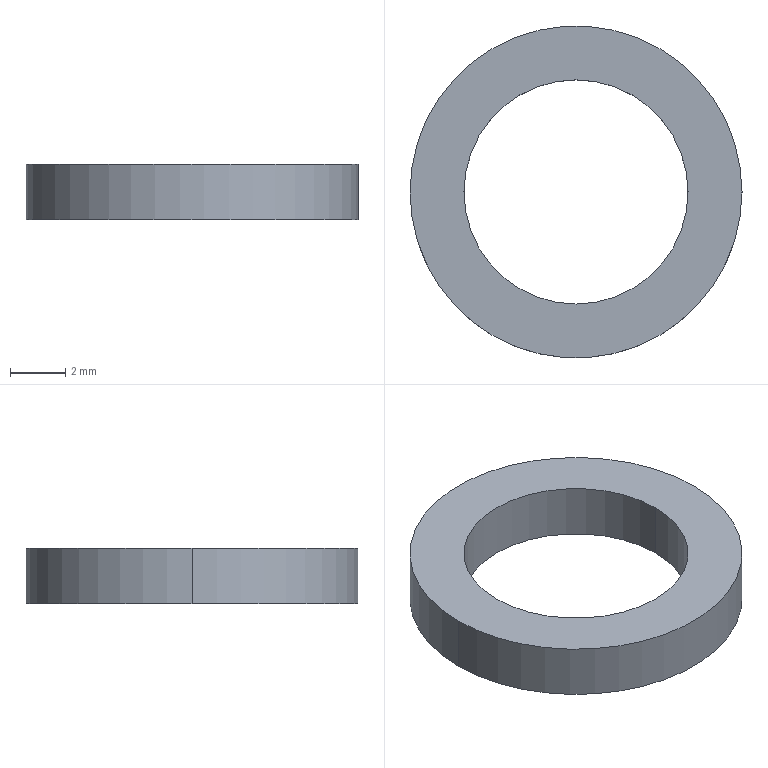Component | SolidWorks | JL001-05-02-1_JL001-05-01-006-1 | 1 solid | 6 faces | box 12 x 12 x 2 mm | volume 123 mm3 | cylinder 4 | plane 2 | commonest cylinder face diameters 8.1 x2 12 x2
build123d program:
from build123d import *

# Parameters (mm, degrees)
SKETCH1_R           = 6
SKETCH1_R_2         = 4.05
BOSS_EXTRUDE1_DEPTH = 2


with BuildPart() as part:
    # Sketch1 → Boss-Extrude1 (new body)
    with BuildSketch(Plane.XY):
        Circle(SKETCH1_R)
        Circle(SKETCH1_R_2, mode=Mode.SUBTRACT)
    extrude(amount=BOSS_EXTRUDE1_DEPTH)


solid = part.part

# Placed as in the assembly
solid = solid.moved(Location((0, 1047.5, 88), (0, 0, 0)))
STEP:
#1=COLOUR_RGB('',0.7922,0.8196,0.9333);
#2=FILL_AREA_STYLE_COLOUR('',#1);
#3=FILL_AREA_STYLE('',(#2));
#4=SURFACE_STYLE_FILL_AREA(#3);
#5=SURFACE_SIDE_STYLE('',(#4));
#6=SURFACE_STYLE_USAGE(.BOTH.,#5);
#7=PRESENTATION_STYLE_ASSIGNMENT((#6));
#8=CARTESIAN_POINT('',(-0.1594,41.24,3.465));
#9=VERTEX_POINT('',#8);
#10=CARTESIAN_POINT('',(0.1594,41.24,3.465));
#11=VERTEX_POINT('',#10);
#12=CARTESIAN_POINT('',(-0.,41.24,3.465));
#13=DIRECTION('',(-0.,0.,-1.));
#14=DIRECTION('',(1.,0.,0.));
#15=AXIS2_PLACEMENT_3D('',#12,#13,#14);
#16=CIRCLE('',#15,0.1594);
#17=EDGE_CURVE('',#9,#11,#16,.T.);
#18=ORIENTED_EDGE('',*,*,#17,.T.);
#19=CARTESIAN_POINT('',(0.1594,41.24,3.543));
#20=VERTEX_POINT('',#19);
#21=CARTESIAN_POINT('',(0.1594,41.24,3.465));
#22=DIRECTION('',(0.,0.,1.));
#23=VECTOR('',#22,39.37);
#24=LINE('',#21,#23);
#25=EDGE_CURVE('',#11,#20,#24,.T.);
#26=ORIENTED_EDGE('',*,*,#25,.T.);
#27=CARTESIAN_POINT('',(-0.1594,41.24,3.543));
#28=VERTEX_POINT('',#27);
#29=CARTESIAN_POINT('',(-0.,41.24,3.543));
#30=DIRECTION('',(-0.,0.,-1.));
#31=DIRECTION('',(1.,0.,0.));
#32=AXIS2_PLACEMENT_3D('',#29,#30,#31);
#33=CIRCLE('',#32,0.1594);
#34=EDGE_CURVE('',#28,#20,#33,.T.);
#35=ORIENTED_EDGE('',*,*,#34,.F.);
#36=CARTESIAN_POINT('',(-0.1594,41.24,3.465));
#37=DIRECTION('',(0.,0.,1.));
#38=VECTOR('',#37,39.37);
#39=LINE('',#36,#38);
#40=EDGE_CURVE('',#9,#28,#39,.T.);
#41=ORIENTED_EDGE('',*,*,#40,.F.);
#42=EDGE_LOOP('',(#18,#26,#35,#41));
#43=FACE_OUTER_BOUND('',#42,.T.);
#44=CARTESIAN_POINT('',(-0.,41.24,3.465));
#45=DIRECTION('',(0.,0.,1.));
#46=DIRECTION('',(-1.,0.,0.));
#47=AXIS2_PLACEMENT_3D('',#44,#45,#46);
#48=CYLINDRICAL_SURFACE('',#47,0.1594);
#49=ADVANCED_FACE('',(#43),#48,.F.);
#50=CARTESIAN_POINT('',(0.2362,41.24,3.465));
#51=VERTEX_POINT('',#50);
#52=CARTESIAN_POINT('',(-0.2362,41.24,3.465));
#53=VERTEX_POINT('',#52);
#54=CARTESIAN_POINT('',(-0.,41.24,3.465));
#55=DIRECTION('',(-0.,0.,-1.));
#56=DIRECTION('',(1.,0.,0.));
#57=AXIS2_PLACEMENT_3D('',#54,#55,#56);
#58=CIRCLE('',#57,0.2362);
#59=EDGE_CURVE('',#51,#53,#58,.T.);
#60=ORIENTED_EDGE('',*,*,#59,.F.);
#61=CARTESIAN_POINT('',(0.2362,41.24,3.543));
#62=VERTEX_POINT('',#61);
#63=CARTESIAN_POINT('',(0.2362,41.24,3.465));
#64=DIRECTION('',(0.,0.,1.));
#65=VECTOR('',#64,39.37);
#66=LINE('',#63,#65);
#67=EDGE_CURVE('',#51,#62,#66,.T.);
#68=ORIENTED_EDGE('',*,*,#67,.T.);
#69=CARTESIAN_POINT('',(-0.2362,41.24,3.543));
#70=VERTEX_POINT('',#69);
#71=CARTESIAN_POINT('',(-0.,41.24,3.543));
#72=DIRECTION('',(-0.,0.,-1.));
#73=DIRECTION('',(1.,0.,0.));
#74=AXIS2_PLACEMENT_3D('',#71,#72,#73);
#75=CIRCLE('',#74,0.2362);
#76=EDGE_CURVE('',#62,#70,#75,.T.);
#77=ORIENTED_EDGE('',*,*,#76,.T.);
#78=CARTESIAN_POINT('',(-0.2362,41.24,3.465));
#79=DIRECTION('',(0.,0.,1.));
#80=VECTOR('',#79,39.37);
#81=LINE('',#78,#80);
#82=EDGE_CURVE('',#53,#70,#81,.T.);
#83=ORIENTED_EDGE('',*,*,#82,.F.);
#84=EDGE_LOOP('',(#60,#68,#77,#83));
#85=FACE_OUTER_BOUND('',#84,.T.);
#86=CARTESIAN_POINT('',(-0.,41.24,3.465));
#87=DIRECTION('',(0.,0.,1.));
#88=DIRECTION('',(-1.,0.,0.));
#89=AXIS2_PLACEMENT_3D('',#86,#87,#88);
#90=CYLINDRICAL_SURFACE('',#89,0.2362);
#91=ADVANCED_FACE('',(#85),#90,.T.);
#92=CARTESIAN_POINT('',(-0.,41.24,3.465));
#93=DIRECTION('',(-0.,0.,-1.));
#94=DIRECTION('',(1.,0.,0.));
#95=AXIS2_PLACEMENT_3D('',#92,#93,#94);
#96=CIRCLE('',#95,0.2362);
#97=EDGE_CURVE('',#53,#51,#96,.T.);
#98=ORIENTED_EDGE('',*,*,#97,.T.);
#99=ORIENTED_EDGE('',*,*,#59,.T.);
#100=EDGE_LOOP('',(#98,#99));
#101=FACE_OUTER_BOUND('',#100,.T.);
#102=ORIENTED_EDGE('',*,*,#17,.F.);
#103=CARTESIAN_POINT('',(-0.,41.24,3.465));
#104=DIRECTION('',(-0.,0.,-1.));
#105=DIRECTION('',(1.,0.,0.));
#106=AXIS2_PLACEMENT_3D('',#103,#104,#105);
#107=CIRCLE('',#106,0.1594);
#108=EDGE_CURVE('',#11,#9,#107,.T.);
#109=ORIENTED_EDGE('',*,*,#108,.F.);
#110=EDGE_LOOP('',(#102,#109));
#111=FACE_BOUND('',#110,.T.);
#112=CARTESIAN_POINT('',(-0.,41.24,3.465));
#113=DIRECTION('',(-0.,0.,-1.));
#114=DIRECTION('',(1.,0.,-0.));
#115=AXIS2_PLACEMENT_3D('',#112,#113,#114);
#116=PLANE('',#115);
#117=ADVANCED_FACE('',(#101,#111),#116,.T.);
#118=CARTESIAN_POINT('',(-0.,41.24,3.543));
#119=DIRECTION('',(-0.,0.,-1.));
#120=DIRECTION('',(1.,0.,0.));
#121=AXIS2_PLACEMENT_3D('',#118,#119,#120);
#122=CIRCLE('',#121,0.2362);
#123=EDGE_CURVE('',#70,#62,#122,.T.);
#124=ORIENTED_EDGE('',*,*,#123,.F.);
#125=ORIENTED_EDGE('',*,*,#76,.F.);
#126=EDGE_LOOP('',(#124,#125));
#127=FACE_OUTER_BOUND('',#126,.T.);
#128=ORIENTED_EDGE('',*,*,#34,.T.);
#129=CARTESIAN_POINT('',(-0.,41.24,3.543));
#130=DIRECTION('',(-0.,0.,-1.));
#131=DIRECTION('',(1.,0.,0.));
#132=AXIS2_PLACEMENT_3D('',#129,#130,#131);
#133=CIRCLE('',#132,0.1594);
#134=EDGE_CURVE('',#20,#28,#133,.T.);
#135=ORIENTED_EDGE('',*,*,#134,.T.);
#136=EDGE_LOOP('',(#128,#135));
#137=FACE_BOUND('',#136,.T.);
#138=CARTESIAN_POINT('',(-0.,41.24,3.543));
#139=DIRECTION('',(-0.,0.,-1.));
#140=DIRECTION('',(1.,0.,-0.));
#141=AXIS2_PLACEMENT_3D('',#138,#139,#140);
#142=PLANE('',#141);
#143=ADVANCED_FACE('',(#127,#137),#142,.F.);
#144=ORIENTED_EDGE('',*,*,#67,.F.);
#145=ORIENTED_EDGE('',*,*,#97,.F.);
#146=ORIENTED_EDGE('',*,*,#82,.T.);
#147=ORIENTED_EDGE('',*,*,#123,.T.);
#148=EDGE_LOOP('',(#144,#145,#146,#147));
#149=FACE_OUTER_BOUND('',#148,.T.);
#150=CARTESIAN_POINT('',(-0.,41.24,3.465));
#151=DIRECTION('',(0.,0.,1.));
#152=DIRECTION('',(-1.,0.,0.));
#153=AXIS2_PLACEMENT_3D('',#150,#151,#152);
#154=CYLINDRICAL_SURFACE('',#153,0.2362);
#155=ADVANCED_FACE('',(#149),#154,.T.);
#156=ORIENTED_EDGE('',*,*,#25,.F.);
#157=ORIENTED_EDGE('',*,*,#108,.T.);
#158=ORIENTED_EDGE('',*,*,#40,.T.);
#159=ORIENTED_EDGE('',*,*,#134,.F.);
#160=EDGE_LOOP('',(#156,#157,#158,#159));
#161=FACE_OUTER_BOUND('',#160,.T.);
#162=CARTESIAN_POINT('',(-0.,41.24,3.465));
#163=DIRECTION('',(0.,0.,1.));
#164=DIRECTION('',(-1.,0.,0.));
#165=AXIS2_PLACEMENT_3D('',#162,#163,#164);
#166=CYLINDRICAL_SURFACE('',#165,0.1594);
#167=ADVANCED_FACE('',(#161),#166,.F.);
#168=CLOSED_SHELL('',(#49,#91,#117,#143,#155,#167));
#169=MANIFOLD_SOLID_BREP('',#168);
#170=STYLED_ITEM('',(#7),#169);
#171=(LENGTH_UNIT()NAMED_UNIT(*)SI_UNIT($,.METRE.));
#172=LENGTH_MEASURE_WITH_UNIT(LENGTH_MEASURE(0.0254),#171);
#173=DIMENSIONAL_EXPONENTS(1.,0.,0.,0.,0.,0.,0.);
#174=(CONVERSION_BASED_UNIT('',#172)LENGTH_UNIT()NAMED_UNIT(#173));
#175=UNCERTAINTY_MEASURE_WITH_UNIT(LENGTH_MEASURE(0.00001),#174,'','');
#176=(NAMED_UNIT(*)PLANE_ANGLE_UNIT()SI_UNIT($,.RADIAN.));
#177=(NAMED_UNIT(*)SI_UNIT($,.STERADIAN.)SOLID_ANGLE_UNIT());
#178=(GEOMETRIC_REPRESENTATION_CONTEXT(3)GLOBAL_UNCERTAINTY_ASSIGNED_CONTEXT((#175))GLOBAL_UNIT_ASSIGNED_CONTEXT((#174,#176,#177))REPRESENTATION_CONTEXT('',''));
#179=MECHANICAL_DESIGN_GEOMETRIC_PRESENTATION_REPRESENTATION('',(#170),#178);
#180=CARTESIAN_POINT('',(0.,0.,0.));
#181=DIRECTION('',(0.,0.,1.));
#182=DIRECTION('',(1.,0.,0.));
#183=AXIS2_PLACEMENT_3D('',#180,#181,#182);
#184=(LENGTH_UNIT()NAMED_UNIT(*)SI_UNIT($,.METRE.));
#185=LENGTH_MEASURE_WITH_UNIT(LENGTH_MEASURE(0.0254),#184);
#186=DIMENSIONAL_EXPONENTS(1.,0.,0.,0.,0.,0.,0.);
#187=(CONVERSION_BASED_UNIT('',#185)LENGTH_UNIT()NAMED_UNIT(#186));
#188=UNCERTAINTY_MEASURE_WITH_UNIT(LENGTH_MEASURE(0.00001),#187,'','');
#189=(NAMED_UNIT(*)PLANE_ANGLE_UNIT()SI_UNIT($,.RADIAN.));
#190=(NAMED_UNIT(*)SI_UNIT($,.STERADIAN.)SOLID_ANGLE_UNIT());
#191=(GEOMETRIC_REPRESENTATION_CONTEXT(3)GLOBAL_UNCERTAINTY_ASSIGNED_CONTEXT((#188))GLOBAL_UNIT_ASSIGNED_CONTEXT((#187,#189,#190))REPRESENTATION_CONTEXT('',''));
#192=ADVANCED_BREP_SHAPE_REPRESENTATION('',(#169,#183),#191);
#193=PRESENTATION_LAYER_ASSIGNMENT('','',(#170));